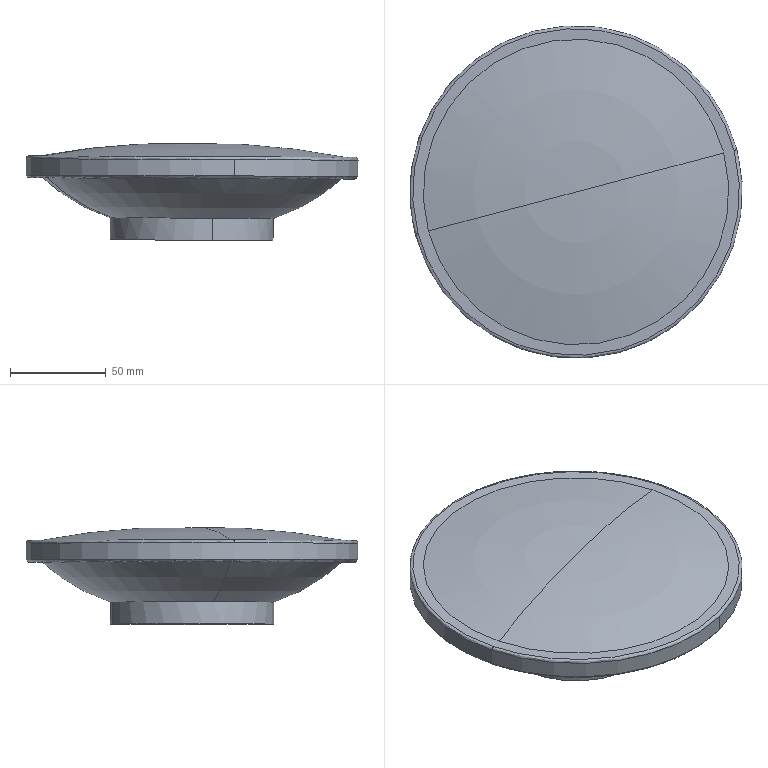Component | SolidWorks | Light-1_RedLight-1 | 1 solid | 15 faces | box 174.03 x 174 x 50.86 mm | volume 678397 mm3 | cylinder 4 | torus 4 | spline 4 | plane 3 | commonest cylinder face diameters 85.497 x2 174 x2
STEP:
#1=COLOUR_RGB('',0.7922,0.8196,0.9333);
#2=FILL_AREA_STYLE_COLOUR('',#1);
#3=FILL_AREA_STYLE('',(#2));
#4=SURFACE_STYLE_FILL_AREA(#3);
#5=SURFACE_SIDE_STYLE('',(#4));
#6=SURFACE_STYLE_USAGE(.BOTH.,#5);
#7=PRESENTATION_STYLE_ASSIGNMENT((#6));
#8=CARTESIAN_POINT('',(-211.965,283.925,12.373));
#9=VERTEX_POINT('',#8);
#10=CARTESIAN_POINT('',(-212.822,287.18,12.377));
#11=VERTEX_POINT('',#10);
#12=CARTESIAN_POINT('',(-212.393,285.552,12.375));
#13=DIRECTION('',(-0.004294,-0.,-1.));
#14=DIRECTION('',(-0.2548,0.967,0.001094));
#15=AXIS2_PLACEMENT_3D('',#12,#13,#14);
#16=CIRCLE('',#15,1.683);
#17=EDGE_CURVE('',#9,#11,#16,.T.);
#18=ORIENTED_EDGE('',*,*,#17,.F.);
#19=CARTESIAN_POINT('',(-211.963,283.925,12.828));
#20=VERTEX_POINT('',#19);
#21=CARTESIAN_POINT('',(-211.965,283.925,12.373));
#22=DIRECTION('',(0.004294,0.,1.));
#23=VECTOR('',#22,39.37);
#24=LINE('',#21,#23);
#25=EDGE_CURVE('',#9,#20,#24,.T.);
#26=ORIENTED_EDGE('',*,*,#25,.T.);
#27=CARTESIAN_POINT('',(-214.019,285.123,12.837));
#28=VERTEX_POINT('',#27);
#29=CARTESIAN_POINT('',(-212.391,285.552,12.83));
#30=DIRECTION('',(0.004294,0.,1.));
#31=DIRECTION('',(0.967,0.2548,-0.004152));
#32=AXIS2_PLACEMENT_3D('',#29,#30,#31);
#33=CIRCLE('',#32,1.683);
#34=EDGE_CURVE('',#28,#20,#33,.T.);
#35=ORIENTED_EDGE('',*,*,#34,.F.);
#36=CARTESIAN_POINT('',(-212.82,287.18,12.832));
#37=VERTEX_POINT('',#36);
#38=CARTESIAN_POINT('',(-212.391,285.552,12.83));
#39=DIRECTION('',(0.004294,0.,1.));
#40=DIRECTION('',(0.967,0.2548,-0.004152));
#41=AXIS2_PLACEMENT_3D('',#38,#39,#40);
#42=CIRCLE('',#41,1.683);
#43=EDGE_CURVE('',#37,#28,#42,.T.);
#44=ORIENTED_EDGE('',*,*,#43,.F.);
#45=CARTESIAN_POINT('',(-212.822,287.18,12.377));
#46=DIRECTION('',(0.004294,0.,1.));
#47=VECTOR('',#46,39.37);
#48=LINE('',#45,#47);
#49=EDGE_CURVE('',#11,#37,#48,.T.);
#50=ORIENTED_EDGE('',*,*,#49,.F.);
#51=EDGE_LOOP('',(#18,#26,#35,#44,#50));
#52=FACE_OUTER_BOUND('',#51,.T.);
#53=CARTESIAN_POINT('',(-212.393,285.552,12.375));
#54=DIRECTION('',(0.004294,0.,1.));
#55=DIRECTION('',(-0.2548,0.967,0.001094));
#56=AXIS2_PLACEMENT_3D('',#53,#54,#55);
#57=CYLINDRICAL_SURFACE('',#56,1.683);
#58=ADVANCED_FACE('',(#52),#57,.T.);
#59=CARTESIAN_POINT('',(-210.764,285.981,12.823));
#60=VERTEX_POINT('',#59);
#61=CARTESIAN_POINT('',(-212.391,285.552,12.83));
#62=DIRECTION('',(0.004294,0.,1.));
#63=DIRECTION('',(0.967,0.2548,-0.004152));
#64=AXIS2_PLACEMENT_3D('',#61,#62,#63);
#65=CIRCLE('',#64,1.683);
#66=EDGE_CURVE('',#60,#37,#65,.T.);
#67=ORIENTED_EDGE('',*,*,#66,.T.);
#68=ORIENTED_EDGE('',*,*,#43,.T.);
#69=CARTESIAN_POINT('',(-215.432,284.75,13.715));
#70=VERTEX_POINT('',#69);
#71=CARTESIAN_POINT('',(-212.869,285.422,16.467));
#72=DIRECTION('',(-0.2548,0.967,0.001094));
#73=DIRECTION('',(-0.967,-0.2548,0.));
#74=AXIS2_PLACEMENT_3D('',#71,#72,#73);
#75=CIRCLE('',#74,3.82);
#76=EDGE_CURVE('',#28,#70,#75,.T.);
#77=ORIENTED_EDGE('',*,*,#76,.T.);
#78=CARTESIAN_POINT('',(-209.343,286.354,13.689));
#79=VERTEX_POINT('',#78);
#80=CARTESIAN_POINT('',(-212.388,285.552,13.702));
#81=DIRECTION('',(-0.004294,-0.,-1.));
#82=DIRECTION('',(0.967,0.2548,-0.004152));
#83=AXIS2_PLACEMENT_3D('',#80,#81,#82);
#84=CIRCLE('',#83,3.148);
#85=EDGE_CURVE('',#70,#79,#84,.T.);
#86=ORIENTED_EDGE('',*,*,#85,.T.);
#87=CARTESIAN_POINT('',(-211.882,285.682,16.463));
#88=DIRECTION('',(0.2548,-0.967,-0.001094));
#89=DIRECTION('',(0.967,0.2548,0.));
#90=AXIS2_PLACEMENT_3D('',#87,#88,#89);
#91=CIRCLE('',#90,3.82);
#92=EDGE_CURVE('',#60,#79,#91,.T.);
#93=ORIENTED_EDGE('',*,*,#92,.F.);
#94=EDGE_LOOP('',(#67,#68,#77,#86,#93));
#95=FACE_OUTER_BOUND('',#94,.T.);
#96=CARTESIAN_POINT('',(-212.376,285.552,16.465));
#97=DIRECTION('',(0.004294,0.,1.));
#98=DIRECTION('',(0.967,0.2548,-0.004152));
#99=AXIS2_PLACEMENT_3D('',#96,#97,#98);
#100=TOROIDAL_SURFACE('',#99,0.5101,3.82);
#101=ADVANCED_FACE('',(#95),#100,.T.);
#102=CARTESIAN_POINT('',(-211.515,282.24,13.699));
#103=VERTEX_POINT('',#102);
#104=CARTESIAN_POINT('',(-215.7,284.68,13.717));
#105=VERTEX_POINT('',#104);
#106=CARTESIAN_POINT('',(-212.388,285.552,13.702));
#107=DIRECTION('',(-0.004294,-0.,-1.));
#108=DIRECTION('',(-0.967,-0.2548,0.004152));
#109=AXIS2_PLACEMENT_3D('',#106,#107,#108);
#110=CIRCLE('',#109,3.425);
#111=EDGE_CURVE('',#103,#105,#110,.T.);
#112=ORIENTED_EDGE('',*,*,#111,.F.);
#113=CARTESIAN_POINT('',(-211.514,282.24,14.033));
#114=VERTEX_POINT('',#113);
#115=CARTESIAN_POINT('',(-211.515,282.24,13.699));
#116=DIRECTION('',(0.004294,0.,1.));
#117=VECTOR('',#116,39.37);
#118=LINE('',#115,#117);
#119=EDGE_CURVE('',#103,#114,#118,.T.);
#120=ORIENTED_EDGE('',*,*,#119,.T.);
#121=CARTESIAN_POINT('',(-215.698,284.68,14.051));
#122=VERTEX_POINT('',#121);
#123=CARTESIAN_POINT('',(-212.386,285.552,14.037));
#124=DIRECTION('',(0.004294,0.,1.));
#125=DIRECTION('',(0.967,0.2548,-0.004152));
#126=AXIS2_PLACEMENT_3D('',#123,#124,#125);
#127=CIRCLE('',#126,3.425);
#128=EDGE_CURVE('',#122,#114,#127,.T.);
#129=ORIENTED_EDGE('',*,*,#128,.F.);
#130=CARTESIAN_POINT('',(-213.259,288.864,14.041));
#131=VERTEX_POINT('',#130);
#132=CARTESIAN_POINT('',(-212.386,285.552,14.037));
#133=DIRECTION('',(0.004294,0.,1.));
#134=DIRECTION('',(0.967,0.2548,-0.004152));
#135=AXIS2_PLACEMENT_3D('',#132,#133,#134);
#136=CIRCLE('',#135,3.425);
#137=EDGE_CURVE('',#131,#122,#136,.T.);
#138=ORIENTED_EDGE('',*,*,#137,.F.);
#139=CARTESIAN_POINT('',(-213.26,288.864,13.706));
#140=VERTEX_POINT('',#139);
#141=CARTESIAN_POINT('',(-213.26,288.864,13.706));
#142=DIRECTION('',(0.004294,0.,1.));
#143=VECTOR('',#142,39.37);
#144=LINE('',#141,#143);
#145=EDGE_CURVE('',#140,#131,#144,.T.);
#146=ORIENTED_EDGE('',*,*,#145,.F.);
#147=CARTESIAN_POINT('',(-212.388,285.552,13.702));
#148=DIRECTION('',(-0.004294,-0.,-1.));
#149=DIRECTION('',(0.967,0.2548,-0.004152));
#150=AXIS2_PLACEMENT_3D('',#147,#148,#149);
#151=CIRCLE('',#150,3.425);
#152=EDGE_CURVE('',#105,#140,#151,.T.);
#153=ORIENTED_EDGE('',*,*,#152,.F.);
#154=EDGE_LOOP('',(#112,#120,#129,#138,#146,#153));
#155=FACE_OUTER_BOUND('',#154,.T.);
#156=CARTESIAN_POINT('',(-212.388,285.552,13.702));
#157=DIRECTION('',(0.004294,0.,1.));
#158=DIRECTION('',(-0.2548,0.967,0.001094));
#159=AXIS2_PLACEMENT_3D('',#156,#157,#158);
#160=CYLINDRICAL_SURFACE('',#159,3.425);
#161=ADVANCED_FACE('',(#155),#160,.T.);
#162=CARTESIAN_POINT('',(-215.43,284.75,14.109));
#163=VERTEX_POINT('',#162);
#164=CARTESIAN_POINT('',(-209.342,286.354,14.083));
#165=VERTEX_POINT('',#164);
#166=CARTESIAN_POINT('',(-212.386,285.552,14.096));
#167=DIRECTION('',(-0.004294,-0.,-1.));
#168=DIRECTION('',(0.967,0.2548,-0.004152));
#169=AXIS2_PLACEMENT_3D('',#166,#167,#168);
#170=CIRCLE('',#169,3.148);
#171=EDGE_CURVE('',#163,#165,#170,.T.);
#172=ORIENTED_EDGE('',*,*,#171,.F.);
#173=CARTESIAN_POINT('',(-212.385,285.552,14.366));
#174=VERTEX_POINT('',#173);
#175=CARTESIAN_POINT('',(-212.729,285.478,-0.7282));
#176=DIRECTION('',(-0.2548,0.967,0.001094));
#177=DIRECTION('',(-0.967,-0.2548,0.));
#178=AXIS2_PLACEMENT_3D('',#175,#176,#177);
#179=CIRCLE('',#178,15.099);
#180=EDGE_CURVE('',#163,#174,#179,.T.);
#181=ORIENTED_EDGE('',*,*,#180,.T.);
#182=CARTESIAN_POINT('',(-212.17,285.626,-0.7306));
#183=DIRECTION('',(0.2548,-0.967,-0.001094));
#184=DIRECTION('',(0.967,0.2548,0.));
#185=AXIS2_PLACEMENT_3D('',#182,#183,#184);
#186=CIRCLE('',#185,15.099);
#187=EDGE_CURVE('',#165,#174,#186,.T.);
#188=ORIENTED_EDGE('',*,*,#187,.F.);
#189=EDGE_LOOP('',(#172,#181,#188));
#190=FACE_OUTER_BOUND('',#189,.T.);
#191=CARTESIAN_POINT('',(-212.45,285.552,-0.7294));
#192=DIRECTION('',(0.004294,0.,1.));
#193=DIRECTION('',(0.967,0.2548,-0.004152));
#194=AXIS2_PLACEMENT_3D('',#191,#192,#193);
#195=TOROIDAL_SURFACE('',#194,0.2891,15.099);
#196=ADVANCED_FACE('',(#190),#195,.T.);
#197=ORIENTED_EDGE('',*,*,#25,.F.);
#198=CARTESIAN_POINT('',(-212.393,285.552,12.375));
#199=DIRECTION('',(-0.004294,-0.,-1.));
#200=DIRECTION('',(-0.2548,0.967,0.001094));
#201=AXIS2_PLACEMENT_3D('',#198,#199,#200);
#202=CIRCLE('',#201,1.683);
#203=EDGE_CURVE('',#11,#9,#202,.T.);
#204=ORIENTED_EDGE('',*,*,#203,.F.);
#205=ORIENTED_EDGE('',*,*,#49,.T.);
#206=ORIENTED_EDGE('',*,*,#66,.F.);
#207=CARTESIAN_POINT('',(-212.391,285.552,12.83));
#208=DIRECTION('',(0.004294,0.,1.));
#209=DIRECTION('',(0.967,0.2548,-0.004152));
#210=AXIS2_PLACEMENT_3D('',#207,#208,#209);
#211=CIRCLE('',#210,1.683);
#212=EDGE_CURVE('',#20,#60,#211,.T.);
#213=ORIENTED_EDGE('',*,*,#212,.F.);
#214=EDGE_LOOP('',(#197,#204,#205,#206,#213));
#215=FACE_OUTER_BOUND('',#214,.T.);
#216=CARTESIAN_POINT('',(-212.393,285.552,12.375));
#217=DIRECTION('',(0.004294,0.,1.));
#218=DIRECTION('',(-0.2548,0.967,0.001094));
#219=AXIS2_PLACEMENT_3D('',#216,#217,#218);
#220=CYLINDRICAL_SURFACE('',#219,1.683);
#221=ADVANCED_FACE('',(#215),#220,.T.);
#222=ORIENTED_EDGE('',*,*,#203,.T.);
#223=ORIENTED_EDGE('',*,*,#17,.T.);
#224=EDGE_LOOP('',(#222,#223));
#225=FACE_OUTER_BOUND('',#224,.T.);
#226=CARTESIAN_POINT('',(-210.312,284.339,12.366));
#227=DIRECTION('',(-0.004294,-0.,-1.));
#228=DIRECTION('',(-0.967,-0.2548,0.004152));
#229=AXIS2_PLACEMENT_3D('',#226,#227,#228);
#230=PLANE('',#229);
#231=ADVANCED_FACE('',(#225),#230,.T.);
#232=ORIENTED_EDGE('',*,*,#76,.F.);
#233=ORIENTED_EDGE('',*,*,#34,.T.);
#234=ORIENTED_EDGE('',*,*,#212,.T.);
#235=ORIENTED_EDGE('',*,*,#92,.T.);
#236=CARTESIAN_POINT('',(-212.388,285.552,13.702));
#237=DIRECTION('',(-0.004294,-0.,-1.));
#238=DIRECTION('',(0.967,0.2548,-0.004152));
#239=AXIS2_PLACEMENT_3D('',#236,#237,#238);
#240=CIRCLE('',#239,3.148);
#241=EDGE_CURVE('',#79,#70,#240,.T.);
#242=ORIENTED_EDGE('',*,*,#241,.T.);
#243=EDGE_LOOP('',(#232,#233,#234,#235,#242));
#244=FACE_OUTER_BOUND('',#243,.T.);
#245=CARTESIAN_POINT('',(-212.376,285.552,16.465));
#246=DIRECTION('',(0.004294,0.,1.));
#247=DIRECTION('',(0.967,0.2548,-0.004152));
#248=AXIS2_PLACEMENT_3D('',#245,#246,#247);
#249=TOROIDAL_SURFACE('',#248,0.5101,3.82);
#250=ADVANCED_FACE('',(#244),#249,.T.);
#251=ORIENTED_EDGE('',*,*,#241,.F.);
#252=ORIENTED_EDGE('',*,*,#85,.F.);
#253=EDGE_LOOP('',(#251,#252));
#254=FACE_BOUND('',#253,.T.);
#255=CARTESIAN_POINT('',(-215.522,284.726,13.716));
#256=VERTEX_POINT('',#255);
#257=CARTESIAN_POINT('',(-209.253,286.378,13.689));
#258=VERTEX_POINT('',#257);
#259=CARTESIAN_POINT('',(-215.522,284.726,13.716));
#260=CARTESIAN_POINT('',(-217.173,290.995,13.723));
#261=CARTESIAN_POINT('',(-210.905,292.646,13.696));
#262=CARTESIAN_POINT('',(-209.253,286.378,13.689));
#263=(BOUNDED_CURVE()B_SPLINE_CURVE(3,(#259,#260,#261,#262),.UNSPECIFIED.,.F.,.F.)B_SPLINE_CURVE_WITH_KNOTS((4,4),(0.,0.259),.UNSPECIFIED.)CURVE()GEOMETRIC_REPRESENTATION_ITEM()RATIONAL_B_SPLINE_CURVE((0.9366,0.3122,0.3122,0.9366))REPRESENTATION_ITEM(''));
#264=EDGE_CURVE('',#256,#258,#263,.T.);
#265=ORIENTED_EDGE('',*,*,#264,.T.);
#266=CARTESIAN_POINT('',(-209.253,286.378,13.689));
#267=CARTESIAN_POINT('',(-207.602,280.109,13.682));
#268=CARTESIAN_POINT('',(-213.87,278.458,13.709));
#269=CARTESIAN_POINT('',(-215.522,284.726,13.716));
#270=(BOUNDED_CURVE()B_SPLINE_CURVE(3,(#266,#267,#268,#269),.UNSPECIFIED.,.F.,.T.)B_SPLINE_CURVE_WITH_KNOTS((4,4),(0.,0.259),.UNSPECIFIED.)CURVE()GEOMETRIC_REPRESENTATION_ITEM()RATIONAL_B_SPLINE_CURVE((0.9366,0.3122,0.3122,0.9366))REPRESENTATION_ITEM(''));
#271=EDGE_CURVE('',#258,#256,#270,.T.);
#272=ORIENTED_EDGE('',*,*,#271,.T.);
#273=EDGE_LOOP('',(#265,#272));
#274=FACE_OUTER_BOUND('',#273,.T.);
#275=CARTESIAN_POINT('',(-208.38,283.216,13.685));
#276=DIRECTION('',(-0.004294,-0.,-1.));
#277=DIRECTION('',(-0.967,-0.2548,0.004152));
#278=AXIS2_PLACEMENT_3D('',#275,#276,#277);
#279=PLANE('',#278);
#280=ADVANCED_FACE('',(#254,#274),#279,.T.);
#281=CARTESIAN_POINT('',(-209.075,286.425,13.688));
#282=VERTEX_POINT('',#281);
#283=CARTESIAN_POINT('',(-209.253,286.378,13.689));
#284=CARTESIAN_POINT('',(-209.212,286.389,13.602));
#285=CARTESIAN_POINT('',(-209.118,286.414,13.601));
#286=CARTESIAN_POINT('',(-209.075,286.425,13.688));
#287=(BOUNDED_CURVE()B_SPLINE_CURVE(3,(#283,#284,#285,#286),.UNSPECIFIED.,.F.,.T.)B_SPLINE_CURVE_WITH_KNOTS((4,4),(0.05172,0.9483),.UNSPECIFIED.)CURVE()GEOMETRIC_REPRESENTATION_ITEM()RATIONAL_B_SPLINE_CURVE((0.9366,0.5904,0.5904,0.9366))REPRESENTATION_ITEM(''));
#288=EDGE_CURVE('',#258,#282,#287,.T.);
#289=ORIENTED_EDGE('',*,*,#288,.T.);
#290=CARTESIAN_POINT('',(-212.388,285.552,13.702));
#291=DIRECTION('',(-0.004294,-0.,-1.));
#292=DIRECTION('',(-0.967,-0.2548,0.004152));
#293=AXIS2_PLACEMENT_3D('',#290,#291,#292);
#294=CIRCLE('',#293,3.425);
#295=EDGE_CURVE('',#282,#103,#294,.T.);
#296=ORIENTED_EDGE('',*,*,#295,.T.);
#297=ORIENTED_EDGE('',*,*,#111,.T.);
#298=CARTESIAN_POINT('',(-215.7,284.68,13.717));
#299=CARTESIAN_POINT('',(-215.658,284.691,13.629));
#300=CARTESIAN_POINT('',(-215.564,284.715,13.629));
#301=CARTESIAN_POINT('',(-215.522,284.726,13.716));
#302=(BOUNDED_CURVE()B_SPLINE_CURVE(3,(#298,#299,#300,#301),.UNSPECIFIED.,.F.,.F.)B_SPLINE_CURVE_WITH_KNOTS((4,4),(0.05172,0.9483),.UNSPECIFIED.)CURVE()GEOMETRIC_REPRESENTATION_ITEM()RATIONAL_B_SPLINE_CURVE((0.9366,0.5904,0.5904,0.9366))REPRESENTATION_ITEM(''));
#303=EDGE_CURVE('',#105,#256,#302,.T.);
#304=ORIENTED_EDGE('',*,*,#303,.T.);
#305=ORIENTED_EDGE('',*,*,#271,.F.);
#306=EDGE_LOOP('',(#289,#296,#297,#304,#305));
#307=FACE_OUTER_BOUND('',#306,.T.);
#308=CARTESIAN_POINT('',(-215.704,284.678,13.726));
#309=CARTESIAN_POINT('',(-213.956,278.046,13.718));
#310=CARTESIAN_POINT('',(-207.324,279.793,13.69));
#311=CARTESIAN_POINT('',(-209.071,286.426,13.697));
#312=CARTESIAN_POINT('',(-215.666,284.689,13.621));
#313=CARTESIAN_POINT('',(-213.939,278.133,13.613));
#314=CARTESIAN_POINT('',(-207.383,279.86,13.585));
#315=CARTESIAN_POINT('',(-209.11,286.416,13.592));
#316=CARTESIAN_POINT('',(-215.557,284.717,13.62));
#317=CARTESIAN_POINT('',(-213.887,278.38,13.613));
#318=CARTESIAN_POINT('',(-207.55,280.049,13.586));
#319=CARTESIAN_POINT('',(-209.219,286.387,13.593));
#320=CARTESIAN_POINT('',(-215.518,284.727,13.725));
#321=CARTESIAN_POINT('',(-213.868,278.467,13.718));
#322=CARTESIAN_POINT('',(-207.608,280.116,13.691));
#323=CARTESIAN_POINT('',(-209.257,286.377,13.698));
#324=(BOUNDED_SURFACE()B_SPLINE_SURFACE(3,3,((#308,#309,#310,#311),(#312,#313,#314,#315),(#316,#317,#318,#319),(#320,#321,#322,#323)),.UNSPECIFIED.,.F.,.F.,.T.)B_SPLINE_SURFACE_WITH_KNOTS((4,4),(4,4),(0.,1.),(0.,1.),.UNSPECIFIED.)GEOMETRIC_REPRESENTATION_ITEM()RATIONAL_B_SPLINE_SURFACE(((1.,0.3333,0.3333,1.),(0.5693,0.1898,0.1898,0.5693),(0.5693,0.1898,0.1898,0.5693),(1.,0.3333,0.3333,1.)))REPRESENTATION_ITEM('')SURFACE());
#325=ADVANCED_FACE('',(#307),#324,.T.);
#326=ORIENTED_EDGE('',*,*,#152,.T.);
#327=CARTESIAN_POINT('',(-212.388,285.552,13.702));
#328=DIRECTION('',(-0.004294,-0.,-1.));
#329=DIRECTION('',(0.967,0.2548,-0.004152));
#330=AXIS2_PLACEMENT_3D('',#327,#328,#329);
#331=CIRCLE('',#330,3.425);
#332=EDGE_CURVE('',#140,#282,#331,.T.);
#333=ORIENTED_EDGE('',*,*,#332,.T.);
#334=ORIENTED_EDGE('',*,*,#288,.F.);
#335=ORIENTED_EDGE('',*,*,#264,.F.);
#336=ORIENTED_EDGE('',*,*,#303,.F.);
#337=EDGE_LOOP('',(#326,#333,#334,#335,#336));
#338=FACE_OUTER_BOUND('',#337,.T.);
#339=CARTESIAN_POINT('',(-209.071,286.426,13.697));
#340=CARTESIAN_POINT('',(-210.819,293.058,13.705));
#341=CARTESIAN_POINT('',(-217.451,291.311,13.733));
#342=CARTESIAN_POINT('',(-215.704,284.678,13.726));
#343=CARTESIAN_POINT('',(-209.11,286.416,13.592));
#344=CARTESIAN_POINT('',(-210.837,292.971,13.6));
#345=CARTESIAN_POINT('',(-217.393,291.244,13.628));
#346=CARTESIAN_POINT('',(-215.666,284.689,13.621));
#347=CARTESIAN_POINT('',(-209.219,286.387,13.593));
#348=CARTESIAN_POINT('',(-210.889,292.725,13.6));
#349=CARTESIAN_POINT('',(-217.226,291.055,13.627));
#350=CARTESIAN_POINT('',(-215.557,284.717,13.62));
#351=CARTESIAN_POINT('',(-209.257,286.377,13.698));
#352=CARTESIAN_POINT('',(-210.907,292.637,13.705));
#353=CARTESIAN_POINT('',(-217.167,290.988,13.732));
#354=CARTESIAN_POINT('',(-215.518,284.727,13.725));
#355=(BOUNDED_SURFACE()B_SPLINE_SURFACE(3,3,((#339,#340,#341,#342),(#343,#344,#345,#346),(#347,#348,#349,#350),(#351,#352,#353,#354)),.UNSPECIFIED.,.F.,.F.,.F.)B_SPLINE_SURFACE_WITH_KNOTS((4,4),(4,4),(0.,1.),(0.,1.),.UNSPECIFIED.)GEOMETRIC_REPRESENTATION_ITEM()RATIONAL_B_SPLINE_SURFACE(((1.,0.3333,0.3333,1.),(0.5693,0.1898,0.1898,0.5693),(0.5693,0.1898,0.1898,0.5693),(1.,0.3333,0.3333,1.)))REPRESENTATION_ITEM('')SURFACE());
#356=ADVANCED_FACE('',(#338),#355,.T.);
#357=ORIENTED_EDGE('',*,*,#119,.F.);
#358=ORIENTED_EDGE('',*,*,#295,.F.);
#359=ORIENTED_EDGE('',*,*,#332,.F.);
#360=ORIENTED_EDGE('',*,*,#145,.T.);
#361=CARTESIAN_POINT('',(-209.074,286.425,14.023));
#362=VERTEX_POINT('',#361);
#363=CARTESIAN_POINT('',(-212.386,285.552,14.037));
#364=DIRECTION('',(0.004294,0.,1.));
#365=DIRECTION('',(0.967,0.2548,-0.004152));
#366=AXIS2_PLACEMENT_3D('',#363,#364,#365);
#367=CIRCLE('',#366,3.425);
#368=EDGE_CURVE('',#362,#131,#367,.T.);
#369=ORIENTED_EDGE('',*,*,#368,.F.);
#370=CARTESIAN_POINT('',(-212.386,285.552,14.037));
#371=DIRECTION('',(0.004294,0.,1.));
#372=DIRECTION('',(0.967,0.2548,-0.004152));
#373=AXIS2_PLACEMENT_3D('',#370,#371,#372);
#374=CIRCLE('',#373,3.425);
#375=EDGE_CURVE('',#114,#362,#374,.T.);
#376=ORIENTED_EDGE('',*,*,#375,.F.);
#377=EDGE_LOOP('',(#357,#358,#359,#360,#369,#376));
#378=FACE_OUTER_BOUND('',#377,.T.);
#379=CARTESIAN_POINT('',(-212.388,285.552,13.702));
#380=DIRECTION('',(0.004294,0.,1.));
#381=DIRECTION('',(-0.2548,0.967,0.001094));
#382=AXIS2_PLACEMENT_3D('',#379,#380,#381);
#383=CYLINDRICAL_SURFACE('',#382,3.425);
#384=ADVANCED_FACE('',(#378),#383,.T.);
#385=CARTESIAN_POINT('',(-209.131,286.41,14.082));
#386=VERTEX_POINT('',#385);
#387=CARTESIAN_POINT('',(-209.074,286.425,14.023));
#388=CARTESIAN_POINT('',(-209.074,286.425,14.057));
#389=CARTESIAN_POINT('',(-209.097,286.419,14.082));
#390=CARTESIAN_POINT('',(-209.131,286.41,14.082));
#391=(BOUNDED_CURVE()B_SPLINE_CURVE(3,(#387,#388,#389,#390),.UNSPECIFIED.,.F.,.T.)B_SPLINE_CURVE_WITH_KNOTS((4,4),(0.06314,0.9369),.UNSPECIFIED.)CURVE()GEOMETRIC_REPRESENTATION_ITEM()RATIONAL_B_SPLINE_CURVE((0.9566,0.7698,0.7698,0.9566))REPRESENTATION_ITEM(''));
#392=EDGE_CURVE('',#362,#386,#391,.T.);
#393=ORIENTED_EDGE('',*,*,#392,.T.);
#394=CARTESIAN_POINT('',(-215.641,284.695,14.11));
#395=VERTEX_POINT('',#394);
#396=CARTESIAN_POINT('',(-209.131,286.41,14.082));
#397=CARTESIAN_POINT('',(-207.416,279.9,14.075));
#398=CARTESIAN_POINT('',(-213.926,278.184,14.103));
#399=CARTESIAN_POINT('',(-215.641,284.695,14.11));
#400=(BOUNDED_CURVE()B_SPLINE_CURVE(3,(#396,#397,#398,#399),.UNSPECIFIED.,.F.,.F.)B_SPLINE_CURVE_WITH_KNOTS((4,4),(0.,1.),.UNSPECIFIED.)CURVE()GEOMETRIC_REPRESENTATION_ITEM()RATIONAL_B_SPLINE_CURVE((0.9566,0.3189,0.3189,0.9566))REPRESENTATION_ITEM(''));
#401=EDGE_CURVE('',#386,#395,#400,.T.);
#402=ORIENTED_EDGE('',*,*,#401,.T.);
#403=CARTESIAN_POINT('',(-215.641,284.695,14.11));
#404=CARTESIAN_POINT('',(-215.674,284.686,14.11));
#405=CARTESIAN_POINT('',(-215.698,284.68,14.086));
#406=CARTESIAN_POINT('',(-215.698,284.68,14.051));
#407=(BOUNDED_CURVE()B_SPLINE_CURVE(3,(#403,#404,#405,#406),.UNSPECIFIED.,.F.,.F.)B_SPLINE_CURVE_WITH_KNOTS((4,4),(0.06314,0.9369),.UNSPECIFIED.)CURVE()GEOMETRIC_REPRESENTATION_ITEM()RATIONAL_B_SPLINE_CURVE((0.9566,0.7698,0.7698,0.9566))REPRESENTATION_ITEM(''));
#408=EDGE_CURVE('',#395,#122,#407,.T.);
#409=ORIENTED_EDGE('',*,*,#408,.T.);
#410=ORIENTED_EDGE('',*,*,#128,.T.);
#411=ORIENTED_EDGE('',*,*,#375,.T.);
#412=EDGE_LOOP('',(#393,#402,#409,#410,#411));
#413=FACE_OUTER_BOUND('',#412,.T.);
#414=CARTESIAN_POINT('',(-215.635,284.696,14.11));
#415=CARTESIAN_POINT('',(-213.923,278.197,14.102));
#416=CARTESIAN_POINT('',(-207.424,279.909,14.074));
#417=CARTESIAN_POINT('',(-209.137,286.408,14.082));
#418=CARTESIAN_POINT('',(-215.674,284.686,14.114));
#419=CARTESIAN_POINT('',(-213.941,278.109,14.106));
#420=CARTESIAN_POINT('',(-207.365,279.842,14.078));
#421=CARTESIAN_POINT('',(-209.098,286.418,14.086));
#422=CARTESIAN_POINT('',(-215.702,284.679,14.085));
#423=CARTESIAN_POINT('',(-213.955,278.047,14.078));
#424=CARTESIAN_POINT('',(-207.323,279.794,14.049));
#425=CARTESIAN_POINT('',(-209.07,286.426,14.057));
#426=CARTESIAN_POINT('',(-215.698,284.68,14.045));
#427=CARTESIAN_POINT('',(-213.953,278.056,14.038));
#428=CARTESIAN_POINT('',(-207.329,279.801,14.009));
#429=CARTESIAN_POINT('',(-209.074,286.425,14.017));
#430=(BOUNDED_SURFACE()B_SPLINE_SURFACE(3,3,((#414,#415,#416,#417),(#418,#419,#420,#421),(#422,#423,#424,#425),(#426,#427,#428,#429)),.UNSPECIFIED.,.F.,.F.,.T.)B_SPLINE_SURFACE_WITH_KNOTS((4,4),(4,4),(0.,1.),(0.,1.),.UNSPECIFIED.)GEOMETRIC_REPRESENTATION_ITEM()RATIONAL_B_SPLINE_SURFACE(((1.,0.3333,0.3333,1.),(0.7553,0.2518,0.2518,0.7553),(0.7553,0.2518,0.2518,0.7553),(1.,0.3333,0.3333,1.)))REPRESENTATION_ITEM('')SURFACE());
#431=ADVANCED_FACE('',(#413),#430,.T.);
#432=CARTESIAN_POINT('',(-215.641,284.695,14.11));
#433=CARTESIAN_POINT('',(-217.356,291.205,14.117));
#434=CARTESIAN_POINT('',(-210.846,292.92,14.089));
#435=CARTESIAN_POINT('',(-209.131,286.41,14.082));
#436=(BOUNDED_CURVE()B_SPLINE_CURVE(3,(#432,#433,#434,#435),.UNSPECIFIED.,.F.,.T.)B_SPLINE_CURVE_WITH_KNOTS((4,4),(0.,1.),.UNSPECIFIED.)CURVE()GEOMETRIC_REPRESENTATION_ITEM()RATIONAL_B_SPLINE_CURVE((0.9566,0.3189,0.3189,0.9566))REPRESENTATION_ITEM(''));
#437=EDGE_CURVE('',#395,#386,#436,.T.);
#438=ORIENTED_EDGE('',*,*,#437,.T.);
#439=ORIENTED_EDGE('',*,*,#392,.F.);
#440=ORIENTED_EDGE('',*,*,#368,.T.);
#441=ORIENTED_EDGE('',*,*,#137,.T.);
#442=ORIENTED_EDGE('',*,*,#408,.F.);
#443=EDGE_LOOP('',(#438,#439,#440,#441,#442));
#444=FACE_OUTER_BOUND('',#443,.T.);
#445=CARTESIAN_POINT('',(-209.137,286.408,14.082));
#446=CARTESIAN_POINT('',(-210.849,292.907,14.089));
#447=CARTESIAN_POINT('',(-217.347,291.195,14.117));
#448=CARTESIAN_POINT('',(-215.635,284.696,14.11));
#449=CARTESIAN_POINT('',(-209.098,286.418,14.086));
#450=CARTESIAN_POINT('',(-210.83,292.995,14.093));
#451=CARTESIAN_POINT('',(-217.407,291.262,14.121));
#452=CARTESIAN_POINT('',(-215.674,284.686,14.114));
#453=CARTESIAN_POINT('',(-209.07,286.426,14.057));
#454=CARTESIAN_POINT('',(-210.817,293.057,14.064));
#455=CARTESIAN_POINT('',(-217.449,291.31,14.093));
#456=CARTESIAN_POINT('',(-215.702,284.679,14.085));
#457=CARTESIAN_POINT('',(-209.074,286.425,14.017));
#458=CARTESIAN_POINT('',(-210.819,293.048,14.024));
#459=CARTESIAN_POINT('',(-217.443,291.303,14.053));
#460=CARTESIAN_POINT('',(-215.698,284.68,14.045));
#461=(BOUNDED_SURFACE()B_SPLINE_SURFACE(3,3,((#445,#446,#447,#448),(#449,#450,#451,#452),(#453,#454,#455,#456),(#457,#458,#459,#460)),.UNSPECIFIED.,.F.,.F.,.T.)B_SPLINE_SURFACE_WITH_KNOTS((4,4),(4,4),(0.,1.),(0.,1.),.UNSPECIFIED.)GEOMETRIC_REPRESENTATION_ITEM()RATIONAL_B_SPLINE_SURFACE(((1.,0.3333,0.3333,1.),(0.7553,0.2518,0.2518,0.7553),(0.7553,0.2518,0.2518,0.7553),(1.,0.3333,0.3333,1.)))REPRESENTATION_ITEM('')SURFACE());
#462=ADVANCED_FACE('',(#444),#461,.T.);
#463=CARTESIAN_POINT('',(-212.386,285.552,14.096));
#464=DIRECTION('',(-0.004294,-0.,-1.));
#465=DIRECTION('',(0.967,0.2548,-0.004152));
#466=AXIS2_PLACEMENT_3D('',#463,#464,#465);
#467=CIRCLE('',#466,3.148);
#468=EDGE_CURVE('',#165,#163,#467,.T.);
#469=ORIENTED_EDGE('',*,*,#468,.T.);
#470=ORIENTED_EDGE('',*,*,#171,.T.);
#471=EDGE_LOOP('',(#469,#470));
#472=FACE_BOUND('',#471,.T.);
#473=ORIENTED_EDGE('',*,*,#437,.F.);
#474=ORIENTED_EDGE('',*,*,#401,.F.);
#475=EDGE_LOOP('',(#473,#474));
#476=FACE_OUTER_BOUND('',#475,.T.);
#477=CARTESIAN_POINT('',(-214.812,281.39,14.106));
#478=DIRECTION('',(0.004294,0.,1.));
#479=DIRECTION('',(0.967,0.2548,-0.004152));
#480=AXIS2_PLACEMENT_3D('',#477,#478,#479);
#481=PLANE('',#480);
#482=ADVANCED_FACE('',(#472,#476),#481,.T.);
#483=ORIENTED_EDGE('',*,*,#180,.F.);
#484=ORIENTED_EDGE('',*,*,#468,.F.);
#485=ORIENTED_EDGE('',*,*,#187,.T.);
#486=EDGE_LOOP('',(#483,#484,#485));
#487=FACE_OUTER_BOUND('',#486,.T.);
#488=CARTESIAN_POINT('',(-212.45,285.552,-0.7294));
#489=DIRECTION('',(0.004294,0.,1.));
#490=DIRECTION('',(0.967,0.2548,-0.004152));
#491=AXIS2_PLACEMENT_3D('',#488,#489,#490);
#492=TOROIDAL_SURFACE('',#491,0.2891,15.099);
#493=ADVANCED_FACE('',(#487),#492,.T.);
#494=CLOSED_SHELL('',(#58,#101,#161,#196,#221,#231,#250,#280,#325,#356,#384,#431,#462,#482,#493));
#495=MANIFOLD_SOLID_BREP('',#494);
#496=STYLED_ITEM('',(#7),#495);
#497=(LENGTH_UNIT()NAMED_UNIT(*)SI_UNIT($,.METRE.));
#498=LENGTH_MEASURE_WITH_UNIT(LENGTH_MEASURE(0.0254),#497);
#499=DIMENSIONAL_EXPONENTS(1.,0.,0.,0.,0.,0.,0.);
#500=(CONVERSION_BASED_UNIT('',#498)LENGTH_UNIT()NAMED_UNIT(#499));
#501=UNCERTAINTY_MEASURE_WITH_UNIT(LENGTH_MEASURE(0.00001),#500,'','');
#502=(NAMED_UNIT(*)PLANE_ANGLE_UNIT()SI_UNIT($,.RADIAN.));
#503=(NAMED_UNIT(*)SI_UNIT($,.STERADIAN.)SOLID_ANGLE_UNIT());
#504=(GEOMETRIC_REPRESENTATION_CONTEXT(3)GLOBAL_UNCERTAINTY_ASSIGNED_CONTEXT((#501))GLOBAL_UNIT_ASSIGNED_CONTEXT((#500,#502,#503))REPRESENTATION_CONTEXT('',''));
#505=MECHANICAL_DESIGN_GEOMETRIC_PRESENTATION_REPRESENTATION('',(#496),#504);
#506=PRESENTATION_LAYER_ASSIGNMENT('','',(#496));
#507=CARTESIAN_POINT('',(0.,0.,0.));
#508=DIRECTION('',(0.,0.,1.));
#509=DIRECTION('',(1.,0.,0.));
#510=AXIS2_PLACEMENT_3D('',#507,#508,#509);
#511=(LENGTH_UNIT()NAMED_UNIT(*)SI_UNIT($,.METRE.));
#512=LENGTH_MEASURE_WITH_UNIT(LENGTH_MEASURE(0.0254),#511);
#513=DIMENSIONAL_EXPONENTS(1.,0.,0.,0.,0.,0.,0.);
#514=(CONVERSION_BASED_UNIT('',#512)LENGTH_UNIT()NAMED_UNIT(#513));
#515=UNCERTAINTY_MEASURE_WITH_UNIT(LENGTH_MEASURE(0.00001),#514,'','');
#516=(NAMED_UNIT(*)PLANE_ANGLE_UNIT()SI_UNIT($,.RADIAN.));
#517=(NAMED_UNIT(*)SI_UNIT($,.STERADIAN.)SOLID_ANGLE_UNIT());
#518=(GEOMETRIC_REPRESENTATION_CONTEXT(3)GLOBAL_UNCERTAINTY_ASSIGNED_CONTEXT((#515))GLOBAL_UNIT_ASSIGNED_CONTEXT((#514,#516,#517))REPRESENTATION_CONTEXT('',''));
#519=ADVANCED_BREP_SHAPE_REPRESENTATION('',(#495,#510),#518);